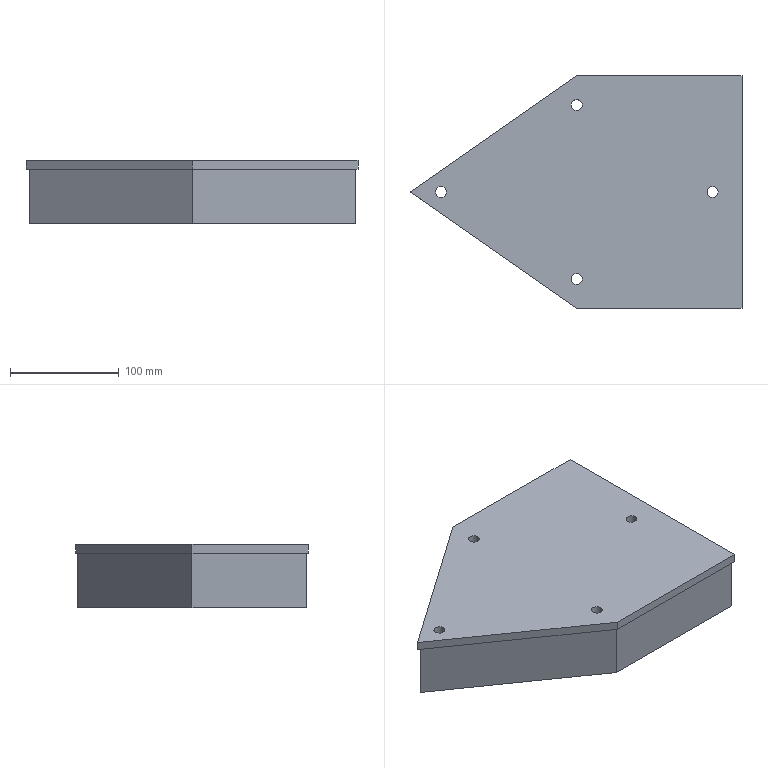Component | NX | EJECTOR_BLOCK | 1 solid | 20 faces | volume 2011493 mm3 | plane 14 | cylinder 4 | other 1 | spline 1 | commonest cylinder face diameters 10.06 x4